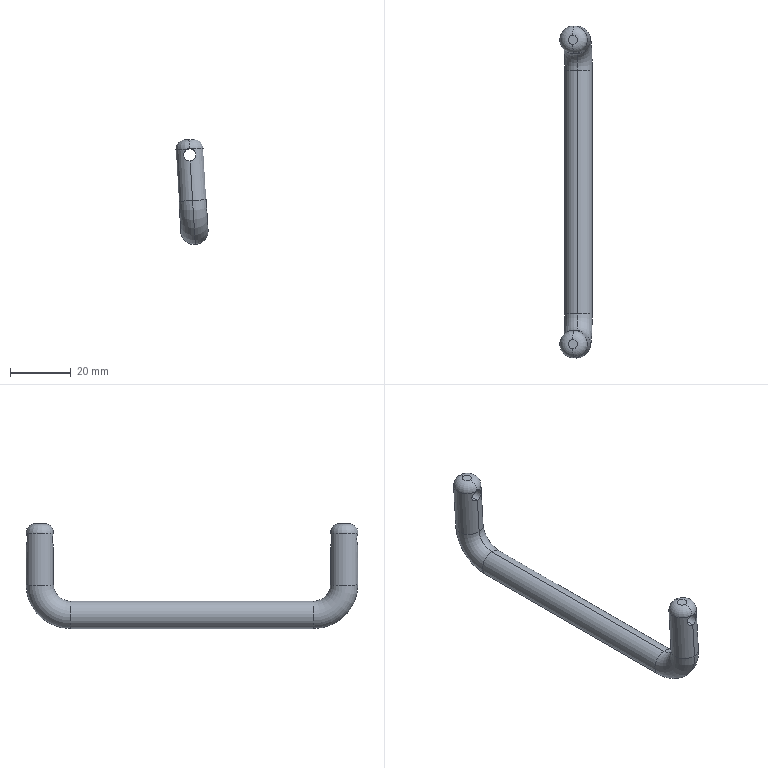Component | SolidWorks | C1-1_C2-1 | 1 solid | 20 faces | box 10.64 x 109 x 34.54 mm | volume 9319 mm3 | cylinder 10 | torus 8 | plane 2 | commonest cylinder face diameters 9 x6 4 x4
build123d program:
from build123d import *

# Parameters (mm, degrees)
SKETCH1_R               = 4.5
FILLET1_R               = 3
CUT_EXTRUDE1_DEPTH      = 111.14
CUT_EXTRUDE1_DEPTH_BACK = 111.14
SKETCH2_R               = 2


with BuildPart() as part:
    # Sweep1: sweep along a curve in space
    with BuildLine() as sweep1_path:
        Line((0, 0, 0), (0, 0, 20))
        ThreePointArc((0, 0, 20), (2.929, 0, 27.071), (10, 0, 30))
        Line((10, 0, 30), (90, 0, 30))
        ThreePointArc((90, 0, 30), (97.071, 0, 27.071), (100, 0, 20))
        Line((100, 0, 20), (100, 0, 0))
    # Sketch1 → Sweep1 (sweep)
    with BuildSketch(Plane.XY):
        Circle(SKETCH1_R)
    sweep(path=sweep1_path.line)

    # Fillet1
    fillet1_edges = [part.edges().sort_by_distance(p)[0] for p in [
        (-4.5, 0, 0),
        (104.5, 0, 0),
    ]]
    fillet(fillet1_edges, radius=FILLET1_R)

    # Sketch2 → Cut-Extrude1 (cut, two sides: drawn at the far end of the back side and taken through both)
    with BuildSketch(Plane(origin=(0, 0, 0), x_dir=(0, 0, -1), z_dir=(1, 0, 0)).offset(-CUT_EXTRUDE1_DEPTH_BACK)):
        with Locations((-5, 0)):
            Circle(SKETCH2_R)
    extrude(amount=CUT_EXTRUDE1_DEPTH + CUT_EXTRUDE1_DEPTH_BACK, mode=Mode.SUBTRACT)


solid = part.part

# Placed as in the assembly
solid = solid.moved(Location((-278.189, -113.128, 595.102), (180, 3.479, -90)))
STEP:
#1=COLOUR_RGB('',0.7922,0.8196,0.9333);
#2=FILL_AREA_STYLE_COLOUR('',#1);
#3=FILL_AREA_STYLE('',(#2));
#4=SURFACE_STYLE_FILL_AREA(#3);
#5=SURFACE_SIDE_STYLE('',(#4));
#6=SURFACE_STYLE_USAGE(.BOTH.,#5);
#7=PRESENTATION_STYLE_ASSIGNMENT((#6));
#8=CARTESIAN_POINT('',(-10.905,-4.277,22.643));
#9=VERTEX_POINT('',#8);
#10=CARTESIAN_POINT('',(-10.905,-4.631,22.643));
#11=VERTEX_POINT('',#10);
#12=CARTESIAN_POINT('',(-10.905,-4.454,22.643));
#13=DIRECTION('',(0.06068,0.,-0.9982));
#14=DIRECTION('',(0.,1.,0.));
#15=AXIS2_PLACEMENT_3D('',#12,#13,#14);
#16=CIRCLE('',#15,0.1772);
#17=EDGE_CURVE('',#9,#11,#16,.T.);
#18=ORIENTED_EDGE('',*,*,#17,.T.);
#19=CARTESIAN_POINT('',(-10.87,-4.06,22.073));
#20=VERTEX_POINT('',#19);
#21=CARTESIAN_POINT('',(-10.905,-4.06,22.643));
#22=DIRECTION('',(0.9982,0.,0.06068));
#23=DIRECTION('',(0.06068,0.,-0.9982));
#24=AXIS2_PLACEMENT_3D('',#21,#22,#23);
#25=CIRCLE('',#24,0.5709);
#26=EDGE_CURVE('',#11,#20,#25,.T.);
#27=ORIENTED_EDGE('',*,*,#26,.T.);
#28=CARTESIAN_POINT('',(-10.891,-4.06,22.427));
#29=VERTEX_POINT('',#28);
#30=CARTESIAN_POINT('',(-10.881,-4.06,22.25));
#31=DIRECTION('',(-0.,1.,0.));
#32=DIRECTION('',(-0.06068,-0.,0.9982));
#33=AXIS2_PLACEMENT_3D('',#30,#31,#32);
#34=CIRCLE('',#33,0.1772);
#35=EDGE_CURVE('',#29,#20,#34,.T.);
#36=ORIENTED_EDGE('',*,*,#35,.F.);
#37=CARTESIAN_POINT('',(-10.905,-4.06,22.643));
#38=DIRECTION('',(0.9982,0.,0.06068));
#39=DIRECTION('',(0.06068,0.,-0.9982));
#40=AXIS2_PLACEMENT_3D('',#37,#38,#39);
#41=CIRCLE('',#40,0.2165);
#42=EDGE_CURVE('',#9,#29,#41,.T.);
#43=ORIENTED_EDGE('',*,*,#42,.F.);
#44=EDGE_LOOP('',(#18,#27,#36,#43));
#45=FACE_OUTER_BOUND('',#44,.T.);
#46=CARTESIAN_POINT('',(-10.905,-4.06,22.643));
#47=DIRECTION('',(0.9982,0.,0.06068));
#48=DIRECTION('',(0.06068,0.,-0.9982));
#49=AXIS2_PLACEMENT_3D('',#46,#47,#48);
#50=TOROIDAL_SURFACE('',#49,0.3937,0.1772);
#51=ADVANCED_FACE('',(#45),#50,.T.);
#52=CARTESIAN_POINT('',(-10.891,-0.9106,22.427));
#53=VERTEX_POINT('',#52);
#54=CARTESIAN_POINT('',(-10.87,-0.9106,22.073));
#55=VERTEX_POINT('',#54);
#56=CARTESIAN_POINT('',(-10.881,-0.9106,22.25));
#57=DIRECTION('',(-0.,1.,0.));
#58=DIRECTION('',(-0.06068,-0.,0.9982));
#59=AXIS2_PLACEMENT_3D('',#56,#57,#58);
#60=CIRCLE('',#59,0.1772);
#61=EDGE_CURVE('',#53,#55,#60,.T.);
#62=ORIENTED_EDGE('',*,*,#61,.T.);
#63=CARTESIAN_POINT('',(-10.905,-0.3397,22.643));
#64=VERTEX_POINT('',#63);
#65=CARTESIAN_POINT('',(-10.905,-0.9106,22.643));
#66=DIRECTION('',(0.9982,0.,0.06068));
#67=DIRECTION('',(0.06068,0.,-0.9982));
#68=AXIS2_PLACEMENT_3D('',#65,#66,#67);
#69=CIRCLE('',#68,0.5709);
#70=EDGE_CURVE('',#55,#64,#69,.T.);
#71=ORIENTED_EDGE('',*,*,#70,.T.);
#72=CARTESIAN_POINT('',(-10.905,-0.694,22.643));
#73=VERTEX_POINT('',#72);
#74=CARTESIAN_POINT('',(-10.905,-0.5169,22.643));
#75=DIRECTION('',(-0.06068,-0.,0.9982));
#76=DIRECTION('',(0.,-1.,0.));
#77=AXIS2_PLACEMENT_3D('',#74,#75,#76);
#78=CIRCLE('',#77,0.1772);
#79=EDGE_CURVE('',#73,#64,#78,.T.);
#80=ORIENTED_EDGE('',*,*,#79,.F.);
#81=CARTESIAN_POINT('',(-10.905,-0.9106,22.643));
#82=DIRECTION('',(0.9982,0.,0.06068));
#83=DIRECTION('',(0.06068,0.,-0.9982));
#84=AXIS2_PLACEMENT_3D('',#81,#82,#83);
#85=CIRCLE('',#84,0.2165);
#86=EDGE_CURVE('',#53,#73,#85,.T.);
#87=ORIENTED_EDGE('',*,*,#86,.F.);
#88=EDGE_LOOP('',(#62,#71,#80,#87));
#89=FACE_OUTER_BOUND('',#88,.T.);
#90=CARTESIAN_POINT('',(-10.905,-0.9106,22.643));
#91=DIRECTION('',(0.9982,0.,0.06068));
#92=DIRECTION('',(0.06068,0.,-0.9982));
#93=AXIS2_PLACEMENT_3D('',#90,#91,#92);
#94=TOROIDAL_SURFACE('',#93,0.3937,0.1772);
#95=ADVANCED_FACE('',(#89),#94,.T.);
#96=CARTESIAN_POINT('',(-10.945,-0.694,23.311));
#97=VERTEX_POINT('',#96);
#98=CARTESIAN_POINT('',(-10.936,-0.694,23.154));
#99=VERTEX_POINT('',#98);
#100=CARTESIAN_POINT('',(-10.945,-0.694,23.311));
#101=CARTESIAN_POINT('',(-10.95,-0.694,23.311));
#102=CARTESIAN_POINT('',(-10.956,-0.6938,23.31));
#103=CARTESIAN_POINT('',(-10.966,-0.6929,23.308));
#104=CARTESIAN_POINT('',(-10.971,-0.6922,23.306));
#105=CARTESIAN_POINT('',(-10.984,-0.6897,23.299));
#106=CARTESIAN_POINT('',(-10.993,-0.6874,23.292));
#107=CARTESIAN_POINT('',(-11.006,-0.6827,23.277));
#108=CARTESIAN_POINT('',(-11.011,-0.6802,23.268));
#109=CARTESIAN_POINT('',(-11.016,-0.6776,23.254));
#110=CARTESIAN_POINT('',(-11.018,-0.6768,23.249));
#111=CARTESIAN_POINT('',(-11.019,-0.6758,23.238));
#112=CARTESIAN_POINT('',(-11.019,-0.6756,23.233));
#113=CARTESIAN_POINT('',(-11.019,-0.6756,23.223));
#114=CARTESIAN_POINT('',(-11.018,-0.6758,23.218));
#115=CARTESIAN_POINT('',(-11.015,-0.6768,23.208));
#116=CARTESIAN_POINT('',(-11.013,-0.6775,23.203));
#117=CARTESIAN_POINT('',(-11.009,-0.6793,23.193));
#118=CARTESIAN_POINT('',(-11.006,-0.6804,23.189));
#119=CARTESIAN_POINT('',(-11.,-0.6826,23.181));
#120=CARTESIAN_POINT('',(-10.996,-0.6839,23.177));
#121=CARTESIAN_POINT('',(-10.989,-0.6862,23.17));
#122=CARTESIAN_POINT('',(-10.985,-0.6874,23.167));
#123=CARTESIAN_POINT('',(-10.976,-0.6896,23.162));
#124=CARTESIAN_POINT('',(-10.971,-0.6906,23.16));
#125=CARTESIAN_POINT('',(-10.957,-0.693,23.155));
#126=CARTESIAN_POINT('',(-10.946,-0.694,23.153));
#127=CARTESIAN_POINT('',(-10.936,-0.694,23.154));
#128=B_SPLINE_CURVE_WITH_KNOTS('',3,(#100,#101,#102,#103,#104,#105,#106,#107,#108,#109,#110,#111,#112,#113,#114,#115,#116,#117,#118,#119,#120,#121,#122,#123,#124,#125,#126,#127),.UNSPECIFIED.,.F.,.F.,(4,2,2,2,2,2,2,2,2,2,2,2,2,4),(0.,0.0003961,0.0007921,0.001584,0.002376,0.002772,0.003168,0.003565,0.003961,0.004357,0.004753,0.005149,0.005545,0.006337),.UNSPECIFIED.);
#129=EDGE_CURVE('',#97,#99,#128,.T.);
#130=ORIENTED_EDGE('',*,*,#129,.T.);
#131=CARTESIAN_POINT('',(-10.936,-0.3397,23.154));
#132=VERTEX_POINT('',#131);
#133=CARTESIAN_POINT('',(-10.936,-4.631,23.154));
#134=DIRECTION('',(-0.,1.,0.));
#135=VECTOR('',#134,39.37);
#136=LINE('',#133,#135);
#137=EDGE_CURVE('',#99,#132,#136,.T.);
#138=ORIENTED_EDGE('',*,*,#137,.T.);
#139=CARTESIAN_POINT('',(-10.945,-0.3397,23.311));
#140=VERTEX_POINT('',#139);
#141=CARTESIAN_POINT('',(-10.936,-0.3397,23.154));
#142=CARTESIAN_POINT('',(-10.941,-0.3397,23.154));
#143=CARTESIAN_POINT('',(-10.946,-0.3399,23.154));
#144=CARTESIAN_POINT('',(-10.956,-0.3408,23.155));
#145=CARTESIAN_POINT('',(-10.961,-0.3415,23.157));
#146=CARTESIAN_POINT('',(-10.976,-0.344,23.162));
#147=CARTESIAN_POINT('',(-10.985,-0.3463,23.167));
#148=CARTESIAN_POINT('',(-10.996,-0.3499,23.177));
#149=CARTESIAN_POINT('',(-11.,-0.3511,23.181));
#150=CARTESIAN_POINT('',(-11.006,-0.3533,23.189));
#151=CARTESIAN_POINT('',(-11.009,-0.3544,23.193));
#152=CARTESIAN_POINT('',(-11.013,-0.3562,23.203));
#153=CARTESIAN_POINT('',(-11.015,-0.3569,23.207));
#154=CARTESIAN_POINT('',(-11.018,-0.3579,23.217));
#155=CARTESIAN_POINT('',(-11.019,-0.3582,23.223));
#156=CARTESIAN_POINT('',(-11.02,-0.3582,23.238));
#157=CARTESIAN_POINT('',(-11.018,-0.3571,23.249));
#158=CARTESIAN_POINT('',(-11.013,-0.3544,23.263));
#159=CARTESIAN_POINT('',(-11.011,-0.3533,23.268));
#160=CARTESIAN_POINT('',(-11.006,-0.3511,23.277));
#161=CARTESIAN_POINT('',(-11.003,-0.3499,23.281));
#162=CARTESIAN_POINT('',(-10.993,-0.3463,23.293));
#163=CARTESIAN_POINT('',(-10.984,-0.344,23.299));
#164=CARTESIAN_POINT('',(-10.97,-0.3415,23.306));
#165=CARTESIAN_POINT('',(-10.966,-0.3408,23.307));
#166=CARTESIAN_POINT('',(-10.956,-0.3399,23.31));
#167=CARTESIAN_POINT('',(-10.95,-0.3397,23.311));
#168=CARTESIAN_POINT('',(-10.945,-0.3397,23.311));
#169=B_SPLINE_CURVE_WITH_KNOTS('',3,(#141,#142,#143,#144,#145,#146,#147,#148,#149,#150,#151,#152,#153,#154,#155,#156,#157,#158,#159,#160,#161,#162,#163,#164,#165,#166,#167,#168),.UNSPECIFIED.,.F.,.F.,(4,2,2,2,2,2,2,2,2,2,2,2,2,4),(0.006337,0.006733,0.007128,0.007919,0.008315,0.008711,0.009106,0.009502,0.01029,0.01069,0.01108,0.01188,0.01227,0.01267),.UNSPECIFIED.);
#170=EDGE_CURVE('',#132,#140,#169,.T.);
#171=ORIENTED_EDGE('',*,*,#170,.T.);
#172=CARTESIAN_POINT('',(-10.945,-4.631,23.311));
#173=DIRECTION('',(-0.,1.,0.));
#174=VECTOR('',#173,39.37);
#175=LINE('',#172,#174);
#176=EDGE_CURVE('',#97,#140,#175,.T.);
#177=ORIENTED_EDGE('',*,*,#176,.F.);
#178=EDGE_LOOP('',(#130,#138,#171,#177));
#179=FACE_OUTER_BOUND('',#178,.T.);
#180=CARTESIAN_POINT('',(-10.94,-4.631,23.233));
#181=DIRECTION('',(-0.,1.,0.));
#182=DIRECTION('',(-0.06068,0.,0.9982));
#183=AXIS2_PLACEMENT_3D('',#180,#181,#182);
#184=CYLINDRICAL_SURFACE('',#183,0.07874);
#185=ADVANCED_FACE('',(#179),#184,.F.);
#186=CARTESIAN_POINT('',(-10.936,-4.631,23.154));
#187=VERTEX_POINT('',#186);
#188=CARTESIAN_POINT('',(-10.945,-4.631,23.311));
#189=VERTEX_POINT('',#188);
#190=CARTESIAN_POINT('',(-10.936,-4.631,23.154));
#191=CARTESIAN_POINT('',(-10.941,-4.631,23.154));
#192=CARTESIAN_POINT('',(-10.946,-4.631,23.154));
#193=CARTESIAN_POINT('',(-10.956,-4.63,23.155));
#194=CARTESIAN_POINT('',(-10.961,-4.629,23.157));
#195=CARTESIAN_POINT('',(-10.976,-4.627,23.162));
#196=CARTESIAN_POINT('',(-10.985,-4.624,23.167));
#197=CARTESIAN_POINT('',(-10.996,-4.621,23.177));
#198=CARTESIAN_POINT('',(-11.,-4.62,23.181));
#199=CARTESIAN_POINT('',(-11.006,-4.617,23.189));
#200=CARTESIAN_POINT('',(-11.009,-4.616,23.193));
#201=CARTESIAN_POINT('',(-11.013,-4.615,23.203));
#202=CARTESIAN_POINT('',(-11.015,-4.614,23.207));
#203=CARTESIAN_POINT('',(-11.018,-4.613,23.217));
#204=CARTESIAN_POINT('',(-11.019,-4.613,23.223));
#205=CARTESIAN_POINT('',(-11.02,-4.613,23.238));
#206=CARTESIAN_POINT('',(-11.018,-4.614,23.249));
#207=CARTESIAN_POINT('',(-11.013,-4.616,23.263));
#208=CARTESIAN_POINT('',(-11.011,-4.617,23.268));
#209=CARTESIAN_POINT('',(-11.006,-4.62,23.277));
#210=CARTESIAN_POINT('',(-11.003,-4.621,23.281));
#211=CARTESIAN_POINT('',(-10.993,-4.624,23.293));
#212=CARTESIAN_POINT('',(-10.984,-4.627,23.299));
#213=CARTESIAN_POINT('',(-10.97,-4.629,23.306));
#214=CARTESIAN_POINT('',(-10.966,-4.63,23.307));
#215=CARTESIAN_POINT('',(-10.956,-4.631,23.31));
#216=CARTESIAN_POINT('',(-10.95,-4.631,23.311));
#217=CARTESIAN_POINT('',(-10.945,-4.631,23.311));
#218=B_SPLINE_CURVE_WITH_KNOTS('',3,(#190,#191,#192,#193,#194,#195,#196,#197,#198,#199,#200,#201,#202,#203,#204,#205,#206,#207,#208,#209,#210,#211,#212,#213,#214,#215,#216,#217),.UNSPECIFIED.,.F.,.F.,(4,2,2,2,2,2,2,2,2,2,2,2,2,4),(0.006337,0.006733,0.007128,0.007919,0.008315,0.008711,0.009106,0.009502,0.01029,0.01069,0.01108,0.01188,0.01227,0.01267),.UNSPECIFIED.);
#219=EDGE_CURVE('',#187,#189,#218,.T.);
#220=ORIENTED_EDGE('',*,*,#219,.F.);
#221=CARTESIAN_POINT('',(-10.936,-4.277,23.154));
#222=VERTEX_POINT('',#221);
#223=CARTESIAN_POINT('',(-10.936,-4.631,23.154));
#224=DIRECTION('',(-0.,1.,0.));
#225=VECTOR('',#224,39.37);
#226=LINE('',#223,#225);
#227=EDGE_CURVE('',#187,#222,#226,.T.);
#228=ORIENTED_EDGE('',*,*,#227,.T.);
#229=CARTESIAN_POINT('',(-10.945,-4.277,23.311));
#230=VERTEX_POINT('',#229);
#231=CARTESIAN_POINT('',(-10.945,-4.277,23.311));
#232=CARTESIAN_POINT('',(-10.95,-4.277,23.311));
#233=CARTESIAN_POINT('',(-10.956,-4.277,23.31));
#234=CARTESIAN_POINT('',(-10.966,-4.278,23.308));
#235=CARTESIAN_POINT('',(-10.971,-4.279,23.306));
#236=CARTESIAN_POINT('',(-10.984,-4.281,23.299));
#237=CARTESIAN_POINT('',(-10.993,-4.283,23.292));
#238=CARTESIAN_POINT('',(-11.006,-4.288,23.277));
#239=CARTESIAN_POINT('',(-11.011,-4.291,23.268));
#240=CARTESIAN_POINT('',(-11.016,-4.293,23.254));
#241=CARTESIAN_POINT('',(-11.018,-4.294,23.249));
#242=CARTESIAN_POINT('',(-11.019,-4.295,23.238));
#243=CARTESIAN_POINT('',(-11.019,-4.295,23.233));
#244=CARTESIAN_POINT('',(-11.019,-4.295,23.223));
#245=CARTESIAN_POINT('',(-11.018,-4.295,23.218));
#246=CARTESIAN_POINT('',(-11.015,-4.294,23.208));
#247=CARTESIAN_POINT('',(-11.013,-4.293,23.203));
#248=CARTESIAN_POINT('',(-11.009,-4.291,23.193));
#249=CARTESIAN_POINT('',(-11.006,-4.29,23.189));
#250=CARTESIAN_POINT('',(-11.,-4.288,23.181));
#251=CARTESIAN_POINT('',(-10.996,-4.287,23.177));
#252=CARTESIAN_POINT('',(-10.989,-4.284,23.17));
#253=CARTESIAN_POINT('',(-10.985,-4.283,23.167));
#254=CARTESIAN_POINT('',(-10.976,-4.281,23.162));
#255=CARTESIAN_POINT('',(-10.971,-4.28,23.16));
#256=CARTESIAN_POINT('',(-10.957,-4.278,23.155));
#257=CARTESIAN_POINT('',(-10.946,-4.277,23.153));
#258=CARTESIAN_POINT('',(-10.936,-4.277,23.154));
#259=B_SPLINE_CURVE_WITH_KNOTS('',3,(#231,#232,#233,#234,#235,#236,#237,#238,#239,#240,#241,#242,#243,#244,#245,#246,#247,#248,#249,#250,#251,#252,#253,#254,#255,#256,#257,#258),.UNSPECIFIED.,.F.,.F.,(4,2,2,2,2,2,2,2,2,2,2,2,2,4),(0.,0.0003961,0.0007921,0.001584,0.002376,0.002772,0.003168,0.003565,0.003961,0.004357,0.004753,0.005149,0.005545,0.006337),.UNSPECIFIED.);
#260=EDGE_CURVE('',#230,#222,#259,.T.);
#261=ORIENTED_EDGE('',*,*,#260,.F.);
#262=CARTESIAN_POINT('',(-10.945,-4.631,23.311));
#263=DIRECTION('',(-0.,1.,0.));
#264=VECTOR('',#263,39.37);
#265=LINE('',#262,#264);
#266=EDGE_CURVE('',#189,#230,#265,.T.);
#267=ORIENTED_EDGE('',*,*,#266,.F.);
#268=EDGE_LOOP('',(#220,#228,#261,#267));
#269=FACE_OUTER_BOUND('',#268,.T.);
#270=CARTESIAN_POINT('',(-10.94,-4.631,23.233));
#271=DIRECTION('',(-0.,1.,0.));
#272=DIRECTION('',(-0.06068,0.,0.9982));
#273=AXIS2_PLACEMENT_3D('',#270,#271,#272);
#274=CYLINDRICAL_SURFACE('',#273,0.07874);
#275=ADVANCED_FACE('',(#269),#274,.F.);
#276=CARTESIAN_POINT('',(-10.945,-0.5169,23.311));
#277=DIRECTION('',(0.06068,0.,-0.9982));
#278=DIRECTION('',(0.,-1.,0.));
#279=AXIS2_PLACEMENT_3D('',#276,#277,#278);
#280=CIRCLE('',#279,0.1772);
#281=EDGE_CURVE('',#140,#97,#280,.T.);
#282=ORIENTED_EDGE('',*,*,#281,.F.);
#283=CARTESIAN_POINT('',(-10.952,-0.4578,23.429));
#284=VERTEX_POINT('',#283);
#285=CARTESIAN_POINT('',(-10.945,-0.4578,23.311));
#286=DIRECTION('',(0.9982,0.,0.06068));
#287=DIRECTION('',(0.06068,0.,-0.9982));
#288=AXIS2_PLACEMENT_3D('',#285,#286,#287);
#289=CIRCLE('',#288,0.1181);
#290=EDGE_CURVE('',#140,#284,#289,.T.);
#291=ORIENTED_EDGE('',*,*,#290,.T.);
#292=CARTESIAN_POINT('',(-10.952,-0.5759,23.429));
#293=VERTEX_POINT('',#292);
#294=CARTESIAN_POINT('',(-10.952,-0.5169,23.429));
#295=DIRECTION('',(-0.06068,-0.,0.9982));
#296=DIRECTION('',(0.,-1.,0.));
#297=AXIS2_PLACEMENT_3D('',#294,#295,#296);
#298=CIRCLE('',#297,0.05906);
#299=EDGE_CURVE('',#293,#284,#298,.T.);
#300=ORIENTED_EDGE('',*,*,#299,.F.);
#301=CARTESIAN_POINT('',(-10.945,-0.5759,23.311));
#302=DIRECTION('',(-0.9982,-0.,-0.06068));
#303=DIRECTION('',(-0.06068,0.,0.9982));
#304=AXIS2_PLACEMENT_3D('',#301,#302,#303);
#305=CIRCLE('',#304,0.1181);
#306=EDGE_CURVE('',#97,#293,#305,.T.);
#307=ORIENTED_EDGE('',*,*,#306,.F.);
#308=EDGE_LOOP('',(#282,#291,#300,#307));
#309=FACE_OUTER_BOUND('',#308,.T.);
#310=CARTESIAN_POINT('',(-10.945,-0.5169,23.311));
#311=DIRECTION('',(-0.06068,-0.,0.9982));
#312=DIRECTION('',(0.,-1.,-0.));
#313=AXIS2_PLACEMENT_3D('',#310,#311,#312);
#314=TOROIDAL_SURFACE('',#313,0.05906,0.1181);
#315=ADVANCED_FACE('',(#309),#314,.T.);
#316=CARTESIAN_POINT('',(-10.952,-4.513,23.429));
#317=VERTEX_POINT('',#316);
#318=CARTESIAN_POINT('',(-10.952,-4.395,23.429));
#319=VERTEX_POINT('',#318);
#320=CARTESIAN_POINT('',(-10.952,-4.454,23.429));
#321=DIRECTION('',(-0.06068,-0.,0.9982));
#322=DIRECTION('',(0.,1.,0.));
#323=AXIS2_PLACEMENT_3D('',#320,#321,#322);
#324=CIRCLE('',#323,0.05906);
#325=EDGE_CURVE('',#317,#319,#324,.T.);
#326=ORIENTED_EDGE('',*,*,#325,.F.);
#327=CARTESIAN_POINT('',(-10.945,-4.513,23.311));
#328=DIRECTION('',(0.9982,0.,0.06068));
#329=DIRECTION('',(0.06068,0.,-0.9982));
#330=AXIS2_PLACEMENT_3D('',#327,#328,#329);
#331=CIRCLE('',#330,0.1181);
#332=EDGE_CURVE('',#317,#189,#331,.T.);
#333=ORIENTED_EDGE('',*,*,#332,.T.);
#334=CARTESIAN_POINT('',(-10.945,-4.454,23.311));
#335=DIRECTION('',(0.06068,0.,-0.9982));
#336=DIRECTION('',(0.,1.,0.));
#337=AXIS2_PLACEMENT_3D('',#334,#335,#336);
#338=CIRCLE('',#337,0.1772);
#339=EDGE_CURVE('',#230,#189,#338,.T.);
#340=ORIENTED_EDGE('',*,*,#339,.F.);
#341=CARTESIAN_POINT('',(-10.945,-4.395,23.311));
#342=DIRECTION('',(-0.9982,-0.,-0.06068));
#343=DIRECTION('',(-0.06068,0.,0.9982));
#344=AXIS2_PLACEMENT_3D('',#341,#342,#343);
#345=CIRCLE('',#344,0.1181);
#346=EDGE_CURVE('',#319,#230,#345,.T.);
#347=ORIENTED_EDGE('',*,*,#346,.F.);
#348=EDGE_LOOP('',(#326,#333,#340,#347));
#349=FACE_OUTER_BOUND('',#348,.T.);
#350=CARTESIAN_POINT('',(-10.945,-4.454,23.311));
#351=DIRECTION('',(0.06068,0.,-0.9982));
#352=DIRECTION('',(-0.,1.,0.));
#353=AXIS2_PLACEMENT_3D('',#350,#351,#352);
#354=TOROIDAL_SURFACE('',#353,0.05906,0.1181);
#355=ADVANCED_FACE('',(#349),#354,.T.);
#356=ORIENTED_EDGE('',*,*,#17,.F.);
#357=CARTESIAN_POINT('',(-10.905,-4.277,22.643));
#358=DIRECTION('',(-0.06068,-0.,0.9982));
#359=VECTOR('',#358,39.37);
#360=LINE('',#357,#359);
#361=EDGE_CURVE('',#9,#222,#360,.T.);
#362=ORIENTED_EDGE('',*,*,#361,.T.);
#363=CARTESIAN_POINT('',(-10.936,-4.277,23.154));
#364=CARTESIAN_POINT('',(-10.93,-4.277,23.154));
#365=CARTESIAN_POINT('',(-10.925,-4.277,23.155));
#366=CARTESIAN_POINT('',(-10.915,-4.278,23.158));
#367=CARTESIAN_POINT('',(-10.91,-4.278,23.16));
#368=CARTESIAN_POINT('',(-10.896,-4.281,23.167));
#369=CARTESIAN_POINT('',(-10.888,-4.283,23.173));
#370=CARTESIAN_POINT('',(-10.878,-4.287,23.184));
#371=CARTESIAN_POINT('',(-10.875,-4.288,23.189));
#372=CARTESIAN_POINT('',(-10.87,-4.29,23.197));
#373=CARTESIAN_POINT('',(-10.868,-4.291,23.202));
#374=CARTESIAN_POINT('',(-10.864,-4.293,23.212));
#375=CARTESIAN_POINT('',(-10.863,-4.294,23.217));
#376=CARTESIAN_POINT('',(-10.862,-4.295,23.227));
#377=CARTESIAN_POINT('',(-10.861,-4.295,23.232));
#378=CARTESIAN_POINT('',(-10.862,-4.295,23.248));
#379=CARTESIAN_POINT('',(-10.865,-4.294,23.258));
#380=CARTESIAN_POINT('',(-10.872,-4.291,23.272));
#381=CARTESIAN_POINT('',(-10.875,-4.29,23.276));
#382=CARTESIAN_POINT('',(-10.881,-4.288,23.285));
#383=CARTESIAN_POINT('',(-10.884,-4.287,23.288));
#384=CARTESIAN_POINT('',(-10.896,-4.283,23.298));
#385=CARTESIAN_POINT('',(-10.905,-4.281,23.304));
#386=CARTESIAN_POINT('',(-10.919,-4.278,23.309));
#387=CARTESIAN_POINT('',(-10.924,-4.278,23.31));
#388=CARTESIAN_POINT('',(-10.935,-4.277,23.311));
#389=CARTESIAN_POINT('',(-10.94,-4.277,23.312));
#390=CARTESIAN_POINT('',(-10.945,-4.277,23.311));
#391=B_SPLINE_CURVE_WITH_KNOTS('',3,(#363,#364,#365,#366,#367,#368,#369,#370,#371,#372,#373,#374,#375,#376,#377,#378,#379,#380,#381,#382,#383,#384,#385,#386,#387,#388,#389,#390),.UNSPECIFIED.,.F.,.F.,(4,2,2,2,2,2,2,2,2,2,2,2,2,4),(0.006337,0.006733,0.007128,0.007919,0.008315,0.008711,0.009106,0.009502,0.01029,0.01069,0.01108,0.01188,0.01227,0.01267),.UNSPECIFIED.);
#392=EDGE_CURVE('',#222,#230,#391,.T.);
#393=ORIENTED_EDGE('',*,*,#392,.T.);
#394=ORIENTED_EDGE('',*,*,#339,.T.);
#395=CARTESIAN_POINT('',(-10.945,-4.631,23.311));
#396=CARTESIAN_POINT('',(-10.94,-4.631,23.312));
#397=CARTESIAN_POINT('',(-10.935,-4.631,23.311));
#398=CARTESIAN_POINT('',(-10.924,-4.63,23.31));
#399=CARTESIAN_POINT('',(-10.919,-4.629,23.309));
#400=CARTESIAN_POINT('',(-10.905,-4.627,23.304));
#401=CARTESIAN_POINT('',(-10.896,-4.624,23.298));
#402=CARTESIAN_POINT('',(-10.881,-4.62,23.285));
#403=CARTESIAN_POINT('',(-10.874,-4.617,23.277));
#404=CARTESIAN_POINT('',(-10.867,-4.615,23.263));
#405=CARTESIAN_POINT('',(-10.866,-4.614,23.258));
#406=CARTESIAN_POINT('',(-10.863,-4.613,23.248));
#407=CARTESIAN_POINT('',(-10.862,-4.613,23.243));
#408=CARTESIAN_POINT('',(-10.861,-4.613,23.232));
#409=CARTESIAN_POINT('',(-10.862,-4.613,23.227));
#410=CARTESIAN_POINT('',(-10.863,-4.614,23.217));
#411=CARTESIAN_POINT('',(-10.864,-4.615,23.212));
#412=CARTESIAN_POINT('',(-10.868,-4.616,23.202));
#413=CARTESIAN_POINT('',(-10.87,-4.617,23.197));
#414=CARTESIAN_POINT('',(-10.875,-4.62,23.188));
#415=CARTESIAN_POINT('',(-10.878,-4.621,23.184));
#416=CARTESIAN_POINT('',(-10.885,-4.623,23.177));
#417=CARTESIAN_POINT('',(-10.889,-4.624,23.173));
#418=CARTESIAN_POINT('',(-10.897,-4.627,23.167));
#419=CARTESIAN_POINT('',(-10.901,-4.628,23.164));
#420=CARTESIAN_POINT('',(-10.915,-4.63,23.158));
#421=CARTESIAN_POINT('',(-10.925,-4.631,23.155));
#422=CARTESIAN_POINT('',(-10.936,-4.631,23.154));
#423=B_SPLINE_CURVE_WITH_KNOTS('',3,(#395,#396,#397,#398,#399,#400,#401,#402,#403,#404,#405,#406,#407,#408,#409,#410,#411,#412,#413,#414,#415,#416,#417,#418,#419,#420,#421,#422),.UNSPECIFIED.,.F.,.F.,(4,2,2,2,2,2,2,2,2,2,2,2,2,4),(0.,0.0003961,0.0007921,0.001584,0.002376,0.002772,0.003168,0.003565,0.003961,0.004357,0.004753,0.005149,0.005545,0.006337),.UNSPECIFIED.);
#424=EDGE_CURVE('',#189,#187,#423,.T.);
#425=ORIENTED_EDGE('',*,*,#424,.T.);
#426=CARTESIAN_POINT('',(-10.905,-4.631,22.643));
#427=DIRECTION('',(-0.06068,-0.,0.9982));
#428=VECTOR('',#427,39.37);
#429=LINE('',#426,#428);
#430=EDGE_CURVE('',#11,#187,#429,.T.);
#431=ORIENTED_EDGE('',*,*,#430,.F.);
#432=EDGE_LOOP('',(#356,#362,#393,#394,#425,#431));
#433=FACE_OUTER_BOUND('',#432,.T.);
#434=CARTESIAN_POINT('',(-10.905,-4.454,22.643));
#435=DIRECTION('',(-0.06068,-0.,0.9982));
#436=DIRECTION('',(0.,-1.,0.));
#437=AXIS2_PLACEMENT_3D('',#434,#435,#436);
#438=CYLINDRICAL_SURFACE('',#437,0.1772);
#439=ADVANCED_FACE('',(#433),#438,.T.);
#440=ORIENTED_EDGE('',*,*,#35,.T.);
#441=CARTESIAN_POINT('',(-10.87,-4.06,22.073));
#442=DIRECTION('',(-0.,1.,0.));
#443=VECTOR('',#442,39.37);
#444=LINE('',#441,#443);
#445=EDGE_CURVE('',#20,#55,#444,.T.);
#446=ORIENTED_EDGE('',*,*,#445,.T.);
#447=ORIENTED_EDGE('',*,*,#61,.F.);
#448=CARTESIAN_POINT('',(-10.891,-4.06,22.427));
#449=DIRECTION('',(-0.,1.,0.));
#450=VECTOR('',#449,39.37);
#451=LINE('',#448,#450);
#452=EDGE_CURVE('',#29,#53,#451,.T.);
#453=ORIENTED_EDGE('',*,*,#452,.F.);
#454=EDGE_LOOP('',(#440,#446,#447,#453));
#455=FACE_OUTER_BOUND('',#454,.T.);
#456=CARTESIAN_POINT('',(-10.881,-4.06,22.25));
#457=DIRECTION('',(-0.,1.,0.));
#458=DIRECTION('',(-0.06068,-0.,0.9982));
#459=AXIS2_PLACEMENT_3D('',#456,#457,#458);
#460=CYLINDRICAL_SURFACE('',#459,0.1772);
#461=ADVANCED_FACE('',(#455),#460,.T.);
#462=ORIENTED_EDGE('',*,*,#79,.T.);
#463=CARTESIAN_POINT('',(-10.905,-0.3397,22.643));
#464=DIRECTION('',(-0.06068,-0.,0.9982));
#465=VECTOR('',#464,39.37);
#466=LINE('',#463,#465);
#467=EDGE_CURVE('',#64,#132,#466,.T.);
#468=ORIENTED_EDGE('',*,*,#467,.T.);
#469=CARTESIAN_POINT('',(-10.945,-0.3397,23.311));
#470=CARTESIAN_POINT('',(-10.94,-0.3397,23.312));
#471=CARTESIAN_POINT('',(-10.935,-0.3399,23.311));
#472=CARTESIAN_POINT('',(-10.924,-0.3408,23.31));
#473=CARTESIAN_POINT('',(-10.919,-0.3415,23.309));
#474=CARTESIAN_POINT('',(-10.905,-0.344,23.304));
#475=CARTESIAN_POINT('',(-10.896,-0.3463,23.298));
#476=CARTESIAN_POINT('',(-10.881,-0.3511,23.285));
#477=CARTESIAN_POINT('',(-10.874,-0.3535,23.277));
#478=CARTESIAN_POINT('',(-10.867,-0.3562,23.263));
#479=CARTESIAN_POINT('',(-10.866,-0.3569,23.258));
#480=CARTESIAN_POINT('',(-10.863,-0.3579,23.248));
#481=CARTESIAN_POINT('',(-10.862,-0.3582,23.243));
#482=CARTESIAN_POINT('',(-10.861,-0.3582,23.232));
#483=CARTESIAN_POINT('',(-10.862,-0.3579,23.227));
#484=CARTESIAN_POINT('',(-10.863,-0.3569,23.217));
#485=CARTESIAN_POINT('',(-10.864,-0.3562,23.212));
#486=CARTESIAN_POINT('',(-10.868,-0.3544,23.202));
#487=CARTESIAN_POINT('',(-10.87,-0.3533,23.197));
#488=CARTESIAN_POINT('',(-10.875,-0.3511,23.188));
#489=CARTESIAN_POINT('',(-10.878,-0.3499,23.184));
#490=CARTESIAN_POINT('',(-10.885,-0.3475,23.177));
#491=CARTESIAN_POINT('',(-10.889,-0.3463,23.173));
#492=CARTESIAN_POINT('',(-10.897,-0.3441,23.167));
#493=CARTESIAN_POINT('',(-10.901,-0.3431,23.164));
#494=CARTESIAN_POINT('',(-10.915,-0.3407,23.158));
#495=CARTESIAN_POINT('',(-10.925,-0.3397,23.155));
#496=CARTESIAN_POINT('',(-10.936,-0.3397,23.154));
#497=B_SPLINE_CURVE_WITH_KNOTS('',3,(#469,#470,#471,#472,#473,#474,#475,#476,#477,#478,#479,#480,#481,#482,#483,#484,#485,#486,#487,#488,#489,#490,#491,#492,#493,#494,#495,#496),.UNSPECIFIED.,.F.,.F.,(4,2,2,2,2,2,2,2,2,2,2,2,2,4),(0.,0.0003961,0.0007921,0.001584,0.002376,0.002772,0.003168,0.003565,0.003961,0.004357,0.004753,0.005149,0.005545,0.006337),.UNSPECIFIED.);
#498=EDGE_CURVE('',#140,#132,#497,.T.);
#499=ORIENTED_EDGE('',*,*,#498,.F.);
#500=ORIENTED_EDGE('',*,*,#281,.T.);
#501=CARTESIAN_POINT('',(-10.936,-0.694,23.154));
#502=CARTESIAN_POINT('',(-10.93,-0.694,23.154));
#503=CARTESIAN_POINT('',(-10.925,-0.6938,23.155));
#504=CARTESIAN_POINT('',(-10.915,-0.6929,23.158));
#505=CARTESIAN_POINT('',(-10.91,-0.6922,23.16));
#506=CARTESIAN_POINT('',(-10.896,-0.6897,23.167));
#507=CARTESIAN_POINT('',(-10.888,-0.6874,23.173));
#508=CARTESIAN_POINT('',(-10.878,-0.6838,23.184));
#509=CARTESIAN_POINT('',(-10.875,-0.6826,23.189));
#510=CARTESIAN_POINT('',(-10.87,-0.6804,23.197));
#511=CARTESIAN_POINT('',(-10.868,-0.6793,23.202));
#512=CARTESIAN_POINT('',(-10.864,-0.6775,23.212));
#513=CARTESIAN_POINT('',(-10.863,-0.6768,23.217));
#514=CARTESIAN_POINT('',(-10.862,-0.6758,23.227));
#515=CARTESIAN_POINT('',(-10.861,-0.6756,23.232));
#516=CARTESIAN_POINT('',(-10.862,-0.6756,23.248));
#517=CARTESIAN_POINT('',(-10.865,-0.6767,23.258));
#518=CARTESIAN_POINT('',(-10.872,-0.6793,23.272));
#519=CARTESIAN_POINT('',(-10.875,-0.6804,23.276));
#520=CARTESIAN_POINT('',(-10.881,-0.6826,23.285));
#521=CARTESIAN_POINT('',(-10.884,-0.6838,23.288));
#522=CARTESIAN_POINT('',(-10.896,-0.6874,23.298));
#523=CARTESIAN_POINT('',(-10.905,-0.6897,23.304));
#524=CARTESIAN_POINT('',(-10.919,-0.6922,23.309));
#525=CARTESIAN_POINT('',(-10.924,-0.6929,23.31));
#526=CARTESIAN_POINT('',(-10.935,-0.6938,23.311));
#527=CARTESIAN_POINT('',(-10.94,-0.694,23.312));
#528=CARTESIAN_POINT('',(-10.945,-0.694,23.311));
#529=B_SPLINE_CURVE_WITH_KNOTS('',3,(#501,#502,#503,#504,#505,#506,#507,#508,#509,#510,#511,#512,#513,#514,#515,#516,#517,#518,#519,#520,#521,#522,#523,#524,#525,#526,#527,#528),.UNSPECIFIED.,.F.,.F.,(4,2,2,2,2,2,2,2,2,2,2,2,2,4),(0.006337,0.006733,0.007128,0.007919,0.008315,0.008711,0.009106,0.009502,0.01029,0.01069,0.01108,0.01188,0.01227,0.01267),.UNSPECIFIED.);
#530=EDGE_CURVE('',#99,#97,#529,.T.);
#531=ORIENTED_EDGE('',*,*,#530,.F.);
#532=CARTESIAN_POINT('',(-10.905,-0.694,22.643));
#533=DIRECTION('',(-0.06068,-0.,0.9982));
#534=VECTOR('',#533,39.37);
#535=LINE('',#532,#534);
#536=EDGE_CURVE('',#73,#99,#535,.T.);
#537=ORIENTED_EDGE('',*,*,#536,.F.);
#538=EDGE_LOOP('',(#462,#468,#499,#500,#531,#537));
#539=FACE_OUTER_BOUND('',#538,.T.);
#540=CARTESIAN_POINT('',(-10.905,-0.5169,22.643));
#541=DIRECTION('',(-0.06068,-0.,0.9982));
#542=DIRECTION('',(0.,-1.,0.));
#543=AXIS2_PLACEMENT_3D('',#540,#541,#542);
#544=CYLINDRICAL_SURFACE('',#543,0.1772);
#545=ADVANCED_FACE('',(#539),#544,.T.);
#546=ORIENTED_EDGE('',*,*,#467,.F.);
#547=CARTESIAN_POINT('',(-10.905,-0.5169,22.643));
#548=DIRECTION('',(-0.06068,-0.,0.9982));
#549=DIRECTION('',(0.,-1.,0.));
#550=AXIS2_PLACEMENT_3D('',#547,#548,#549);
#551=CIRCLE('',#550,0.1772);
#552=EDGE_CURVE('',#64,#73,#551,.T.);
#553=ORIENTED_EDGE('',*,*,#552,.T.);
#554=ORIENTED_EDGE('',*,*,#536,.T.);
#555=ORIENTED_EDGE('',*,*,#129,.F.);
#556=CARTESIAN_POINT('',(-10.945,-0.5169,23.311));
#557=DIRECTION('',(0.06068,0.,-0.9982));
#558=DIRECTION('',(0.,-1.,0.));
#559=AXIS2_PLACEMENT_3D('',#556,#557,#558);
#560=CIRCLE('',#559,0.1772);
#561=EDGE_CURVE('',#97,#140,#560,.T.);
#562=ORIENTED_EDGE('',*,*,#561,.T.);
#563=ORIENTED_EDGE('',*,*,#170,.F.);
#564=EDGE_LOOP('',(#546,#553,#554,#555,#562,#563));
#565=FACE_OUTER_BOUND('',#564,.T.);
#566=CARTESIAN_POINT('',(-10.905,-0.5169,22.643));
#567=DIRECTION('',(-0.06068,-0.,0.9982));
#568=DIRECTION('',(0.,-1.,0.));
#569=AXIS2_PLACEMENT_3D('',#566,#567,#568);
#570=CYLINDRICAL_SURFACE('',#569,0.1772);
#571=ADVANCED_FACE('',(#565),#570,.T.);
#572=ORIENTED_EDGE('',*,*,#70,.F.);
#573=CARTESIAN_POINT('',(-10.881,-0.9106,22.25));
#574=DIRECTION('',(-0.,1.,0.));
#575=DIRECTION('',(-0.06068,-0.,0.9982));
#576=AXIS2_PLACEMENT_3D('',#573,#574,#575);
#577=CIRCLE('',#576,0.1772);
#578=EDGE_CURVE('',#55,#53,#577,.T.);
#579=ORIENTED_EDGE('',*,*,#578,.T.);
#580=ORIENTED_EDGE('',*,*,#86,.T.);
#581=ORIENTED_EDGE('',*,*,#552,.F.);
#582=EDGE_LOOP('',(#572,#579,#580,#581));
#583=FACE_OUTER_BOUND('',#582,.T.);
#584=CARTESIAN_POINT('',(-10.905,-0.9106,22.643));
#585=DIRECTION('',(0.9982,0.,0.06068));
#586=DIRECTION('',(0.06068,0.,-0.9982));
#587=AXIS2_PLACEMENT_3D('',#584,#585,#586);
#588=TOROIDAL_SURFACE('',#587,0.3937,0.1772);
#589=ADVANCED_FACE('',(#583),#588,.T.);
#590=ORIENTED_EDGE('',*,*,#445,.F.);
#591=CARTESIAN_POINT('',(-10.881,-4.06,22.25));
#592=DIRECTION('',(-0.,1.,0.));
#593=DIRECTION('',(-0.06068,-0.,0.9982));
#594=AXIS2_PLACEMENT_3D('',#591,#592,#593);
#595=CIRCLE('',#594,0.1772);
#596=EDGE_CURVE('',#20,#29,#595,.T.);
#597=ORIENTED_EDGE('',*,*,#596,.T.);
#598=ORIENTED_EDGE('',*,*,#452,.T.);
#599=ORIENTED_EDGE('',*,*,#578,.F.);
#600=EDGE_LOOP('',(#590,#597,#598,#599));
#601=FACE_OUTER_BOUND('',#600,.T.);
#602=CARTESIAN_POINT('',(-10.881,-4.06,22.25));
#603=DIRECTION('',(-0.,1.,0.));
#604=DIRECTION('',(-0.06068,-0.,0.9982));
#605=AXIS2_PLACEMENT_3D('',#602,#603,#604);
#606=CYLINDRICAL_SURFACE('',#605,0.1772);
#607=ADVANCED_FACE('',(#601),#606,.T.);
#608=ORIENTED_EDGE('',*,*,#26,.F.);
#609=CARTESIAN_POINT('',(-10.905,-4.454,22.643));
#610=DIRECTION('',(0.06068,0.,-0.9982));
#611=DIRECTION('',(0.,1.,0.));
#612=AXIS2_PLACEMENT_3D('',#609,#610,#611);
#613=CIRCLE('',#612,0.1772);
#614=EDGE_CURVE('',#11,#9,#613,.T.);
#615=ORIENTED_EDGE('',*,*,#614,.T.);
#616=ORIENTED_EDGE('',*,*,#42,.T.);
#617=ORIENTED_EDGE('',*,*,#596,.F.);
#618=EDGE_LOOP('',(#608,#615,#616,#617));
#619=FACE_OUTER_BOUND('',#618,.T.);
#620=CARTESIAN_POINT('',(-10.905,-4.06,22.643));
#621=DIRECTION('',(0.9982,0.,0.06068));
#622=DIRECTION('',(0.06068,0.,-0.9982));
#623=AXIS2_PLACEMENT_3D('',#620,#621,#622);
#624=TOROIDAL_SURFACE('',#623,0.3937,0.1772);
#625=ADVANCED_FACE('',(#619),#624,.T.);
#626=ORIENTED_EDGE('',*,*,#361,.F.);
#627=ORIENTED_EDGE('',*,*,#614,.F.);
#628=ORIENTED_EDGE('',*,*,#430,.T.);
#629=ORIENTED_EDGE('',*,*,#219,.T.);
#630=CARTESIAN_POINT('',(-10.945,-4.454,23.311));
#631=DIRECTION('',(0.06068,0.,-0.9982));
#632=DIRECTION('',(0.,1.,0.));
#633=AXIS2_PLACEMENT_3D('',#630,#631,#632);
#634=CIRCLE('',#633,0.1772);
#635=EDGE_CURVE('',#189,#230,#634,.T.);
#636=ORIENTED_EDGE('',*,*,#635,.T.);
#637=ORIENTED_EDGE('',*,*,#260,.T.);
#638=EDGE_LOOP('',(#626,#627,#628,#629,#636,#637));
#639=FACE_OUTER_BOUND('',#638,.T.);
#640=CARTESIAN_POINT('',(-10.905,-4.454,22.643));
#641=DIRECTION('',(-0.06068,-0.,0.9982));
#642=DIRECTION('',(0.,-1.,0.));
#643=AXIS2_PLACEMENT_3D('',#640,#641,#642);
#644=CYLINDRICAL_SURFACE('',#643,0.1772);
#645=ADVANCED_FACE('',(#639),#644,.T.);
#646=ORIENTED_EDGE('',*,*,#299,.T.);
#647=CARTESIAN_POINT('',(-10.952,-0.5169,23.429));
#648=DIRECTION('',(-0.06068,-0.,0.9982));
#649=DIRECTION('',(0.,-1.,0.));
#650=AXIS2_PLACEMENT_3D('',#647,#648,#649);
#651=CIRCLE('',#650,0.05906);
#652=EDGE_CURVE('',#284,#293,#651,.T.);
#653=ORIENTED_EDGE('',*,*,#652,.T.);
#654=EDGE_LOOP('',(#646,#653));
#655=FACE_OUTER_BOUND('',#654,.T.);
#656=CARTESIAN_POINT('',(-10.952,-0.5169,23.429));
#657=DIRECTION('',(-0.06068,-0.,0.9982));
#658=DIRECTION('',(0.,-1.,-0.));
#659=AXIS2_PLACEMENT_3D('',#656,#657,#658);
#660=PLANE('',#659);
#661=ADVANCED_FACE('',(#655),#660,.T.);
#662=CARTESIAN_POINT('',(-10.952,-4.454,23.429));
#663=DIRECTION('',(-0.06068,-0.,0.9982));
#664=DIRECTION('',(0.,1.,0.));
#665=AXIS2_PLACEMENT_3D('',#662,#663,#664);
#666=CIRCLE('',#665,0.05906);
#667=EDGE_CURVE('',#319,#317,#666,.T.);
#668=ORIENTED_EDGE('',*,*,#667,.T.);
#669=ORIENTED_EDGE('',*,*,#325,.T.);
#670=EDGE_LOOP('',(#668,#669));
#671=FACE_OUTER_BOUND('',#670,.T.);
#672=CARTESIAN_POINT('',(-10.952,-4.454,23.429));
#673=DIRECTION('',(0.06068,0.,-0.9982));
#674=DIRECTION('',(-0.,1.,0.));
#675=AXIS2_PLACEMENT_3D('',#672,#673,#674);
#676=PLANE('',#675);
#677=ADVANCED_FACE('',(#671),#676,.F.);
#678=ORIENTED_EDGE('',*,*,#332,.F.);
#679=ORIENTED_EDGE('',*,*,#667,.F.);
#680=ORIENTED_EDGE('',*,*,#346,.T.);
#681=ORIENTED_EDGE('',*,*,#635,.F.);
#682=EDGE_LOOP('',(#678,#679,#680,#681));
#683=FACE_OUTER_BOUND('',#682,.T.);
#684=CARTESIAN_POINT('',(-10.945,-4.454,23.311));
#685=DIRECTION('',(0.06068,0.,-0.9982));
#686=DIRECTION('',(-0.,1.,0.));
#687=AXIS2_PLACEMENT_3D('',#684,#685,#686);
#688=TOROIDAL_SURFACE('',#687,0.05906,0.1181);
#689=ADVANCED_FACE('',(#683),#688,.T.);
#690=ORIENTED_EDGE('',*,*,#290,.F.);
#691=ORIENTED_EDGE('',*,*,#561,.F.);
#692=ORIENTED_EDGE('',*,*,#306,.T.);
#693=ORIENTED_EDGE('',*,*,#652,.F.);
#694=EDGE_LOOP('',(#690,#691,#692,#693));
#695=FACE_OUTER_BOUND('',#694,.T.);
#696=CARTESIAN_POINT('',(-10.945,-0.5169,23.311));
#697=DIRECTION('',(-0.06068,-0.,0.9982));
#698=DIRECTION('',(0.,-1.,-0.));
#699=AXIS2_PLACEMENT_3D('',#696,#697,#698);
#700=TOROIDAL_SURFACE('',#699,0.05906,0.1181);
#701=ADVANCED_FACE('',(#695),#700,.T.);
#702=ORIENTED_EDGE('',*,*,#227,.F.);
#703=ORIENTED_EDGE('',*,*,#424,.F.);
#704=ORIENTED_EDGE('',*,*,#266,.T.);
#705=ORIENTED_EDGE('',*,*,#392,.F.);
#706=EDGE_LOOP('',(#702,#703,#704,#705));
#707=FACE_OUTER_BOUND('',#706,.T.);
#708=CARTESIAN_POINT('',(-10.94,-4.631,23.233));
#709=DIRECTION('',(-0.,1.,0.));
#710=DIRECTION('',(-0.06068,0.,0.9982));
#711=AXIS2_PLACEMENT_3D('',#708,#709,#710);
#712=CYLINDRICAL_SURFACE('',#711,0.07874);
#713=ADVANCED_FACE('',(#707),#712,.F.);
#714=ORIENTED_EDGE('',*,*,#137,.F.);
#715=ORIENTED_EDGE('',*,*,#530,.T.);
#716=ORIENTED_EDGE('',*,*,#176,.T.);
#717=ORIENTED_EDGE('',*,*,#498,.T.);
#718=EDGE_LOOP('',(#714,#715,#716,#717));
#719=FACE_OUTER_BOUND('',#718,.T.);
#720=CARTESIAN_POINT('',(-10.94,-4.631,23.233));
#721=DIRECTION('',(-0.,1.,0.));
#722=DIRECTION('',(-0.06068,0.,0.9982));
#723=AXIS2_PLACEMENT_3D('',#720,#721,#722);
#724=CYLINDRICAL_SURFACE('',#723,0.07874);
#725=ADVANCED_FACE('',(#719),#724,.F.);
#726=CLOSED_SHELL('',(#51,#95,#185,#275,#315,#355,#439,#461,#545,#571,#589,#607,#625,#645,#661,#677,#689,#701,#713,#725));
#727=MANIFOLD_SOLID_BREP('',#726);
#728=STYLED_ITEM('',(#7),#727);
#729=(LENGTH_UNIT()NAMED_UNIT(*)SI_UNIT($,.METRE.));
#730=LENGTH_MEASURE_WITH_UNIT(LENGTH_MEASURE(0.0254),#729);
#731=DIMENSIONAL_EXPONENTS(1.,0.,0.,0.,0.,0.,0.);
#732=(CONVERSION_BASED_UNIT('',#730)LENGTH_UNIT()NAMED_UNIT(#731));
#733=UNCERTAINTY_MEASURE_WITH_UNIT(LENGTH_MEASURE(0.00001),#732,'','');
#734=(NAMED_UNIT(*)PLANE_ANGLE_UNIT()SI_UNIT($,.RADIAN.));
#735=(NAMED_UNIT(*)SI_UNIT($,.STERADIAN.)SOLID_ANGLE_UNIT());
#736=(GEOMETRIC_REPRESENTATION_CONTEXT(3)GLOBAL_UNCERTAINTY_ASSIGNED_CONTEXT((#733))GLOBAL_UNIT_ASSIGNED_CONTEXT((#732,#734,#735))REPRESENTATION_CONTEXT('',''));
#737=MECHANICAL_DESIGN_GEOMETRIC_PRESENTATION_REPRESENTATION('',(#728),#736);
#738=PRESENTATION_LAYER_ASSIGNMENT('','',(#728));
#739=CARTESIAN_POINT('',(0.,0.,0.));
#740=DIRECTION('',(0.,0.,1.));
#741=DIRECTION('',(1.,0.,0.));
#742=AXIS2_PLACEMENT_3D('',#739,#740,#741);
#743=(LENGTH_UNIT()NAMED_UNIT(*)SI_UNIT($,.METRE.));
#744=LENGTH_MEASURE_WITH_UNIT(LENGTH_MEASURE(0.0254),#743);
#745=DIMENSIONAL_EXPONENTS(1.,0.,0.,0.,0.,0.,0.);
#746=(CONVERSION_BASED_UNIT('',#744)LENGTH_UNIT()NAMED_UNIT(#745));
#747=UNCERTAINTY_MEASURE_WITH_UNIT(LENGTH_MEASURE(0.00001),#746,'','');
#748=(NAMED_UNIT(*)PLANE_ANGLE_UNIT()SI_UNIT($,.RADIAN.));
#749=(NAMED_UNIT(*)SI_UNIT($,.STERADIAN.)SOLID_ANGLE_UNIT());
#750=(GEOMETRIC_REPRESENTATION_CONTEXT(3)GLOBAL_UNCERTAINTY_ASSIGNED_CONTEXT((#747))GLOBAL_UNIT_ASSIGNED_CONTEXT((#746,#748,#749))REPRESENTATION_CONTEXT('',''));
#751=ADVANCED_BREP_SHAPE_REPRESENTATION('',(#727,#742),#750);